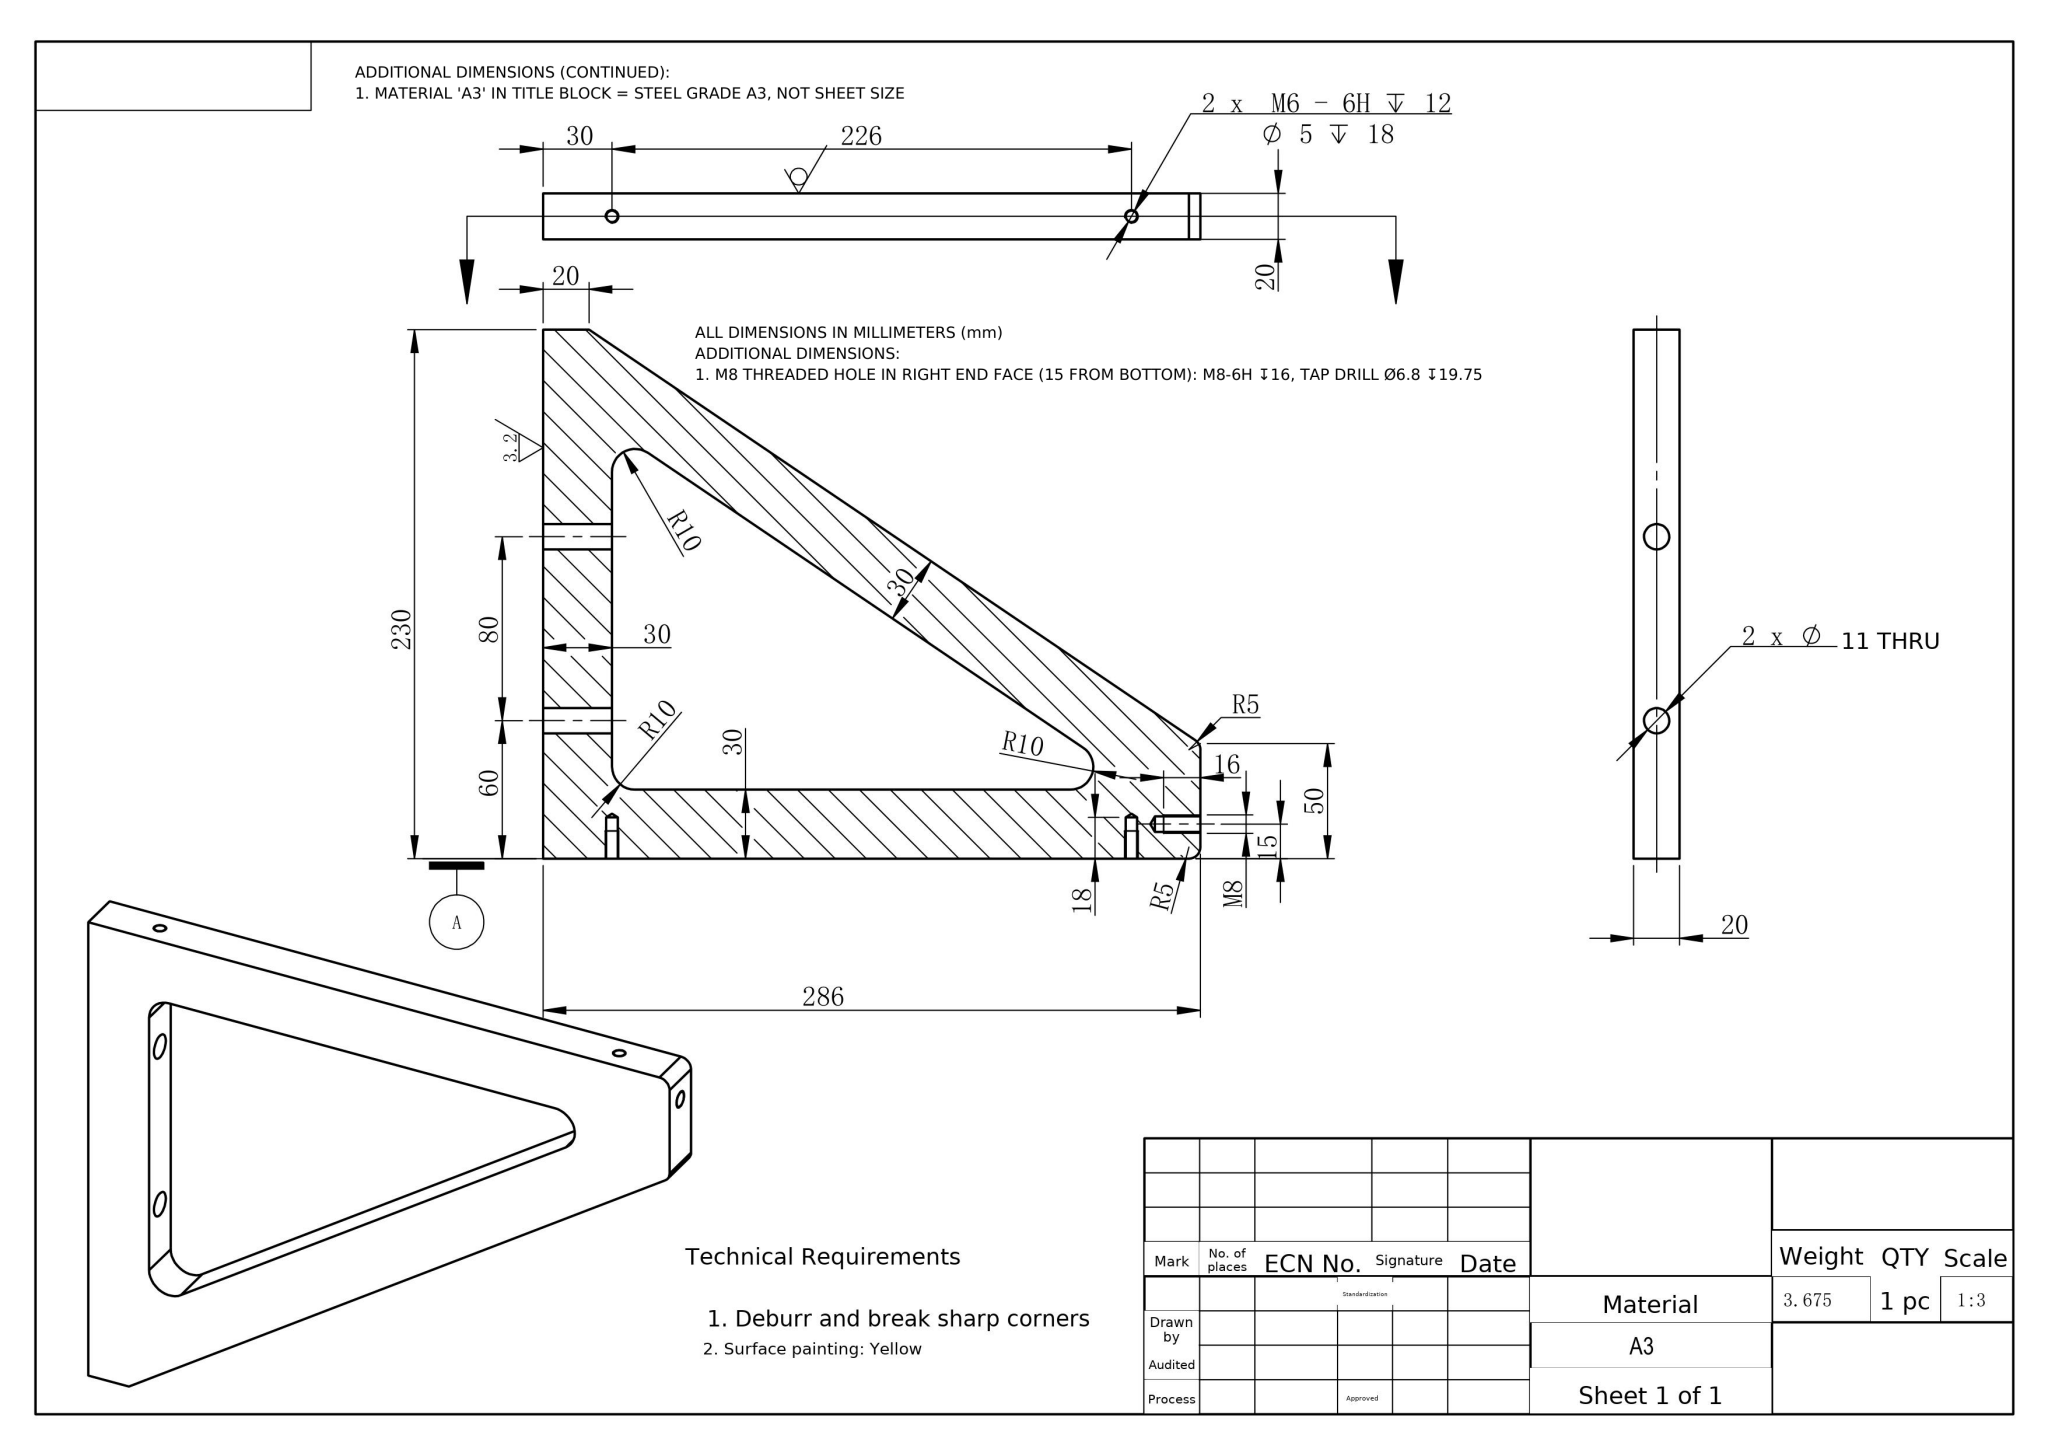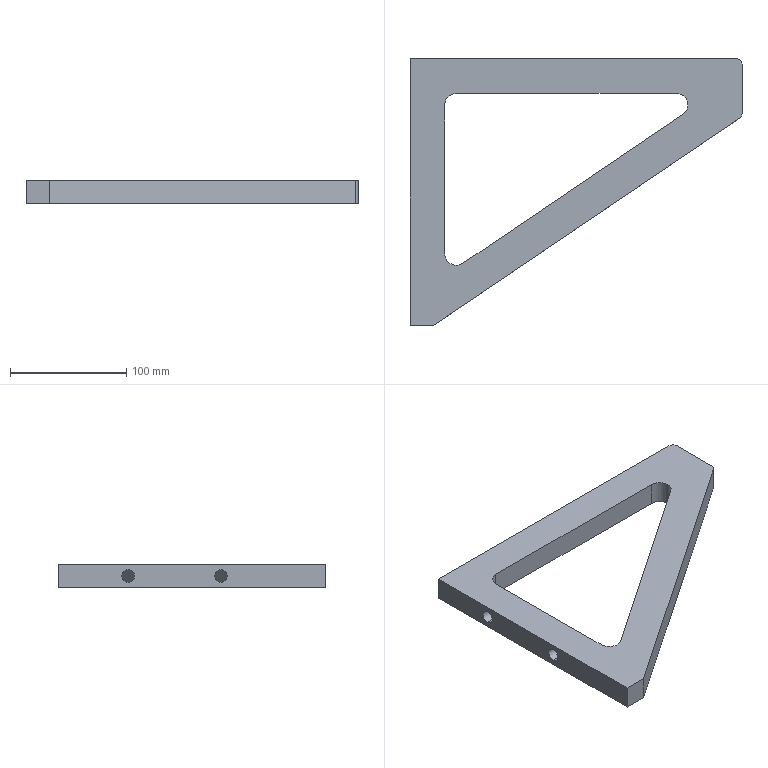Part | NX | mm | 1 solid | 32 faces | box 286 x 230 x 20 mm | volume 471207 mm3 | cylinder 16 | plane 10 | cone 6 | commonest cylinder face diameters 5 x4 11 x4 20 x4 6.8 x2 10 x2